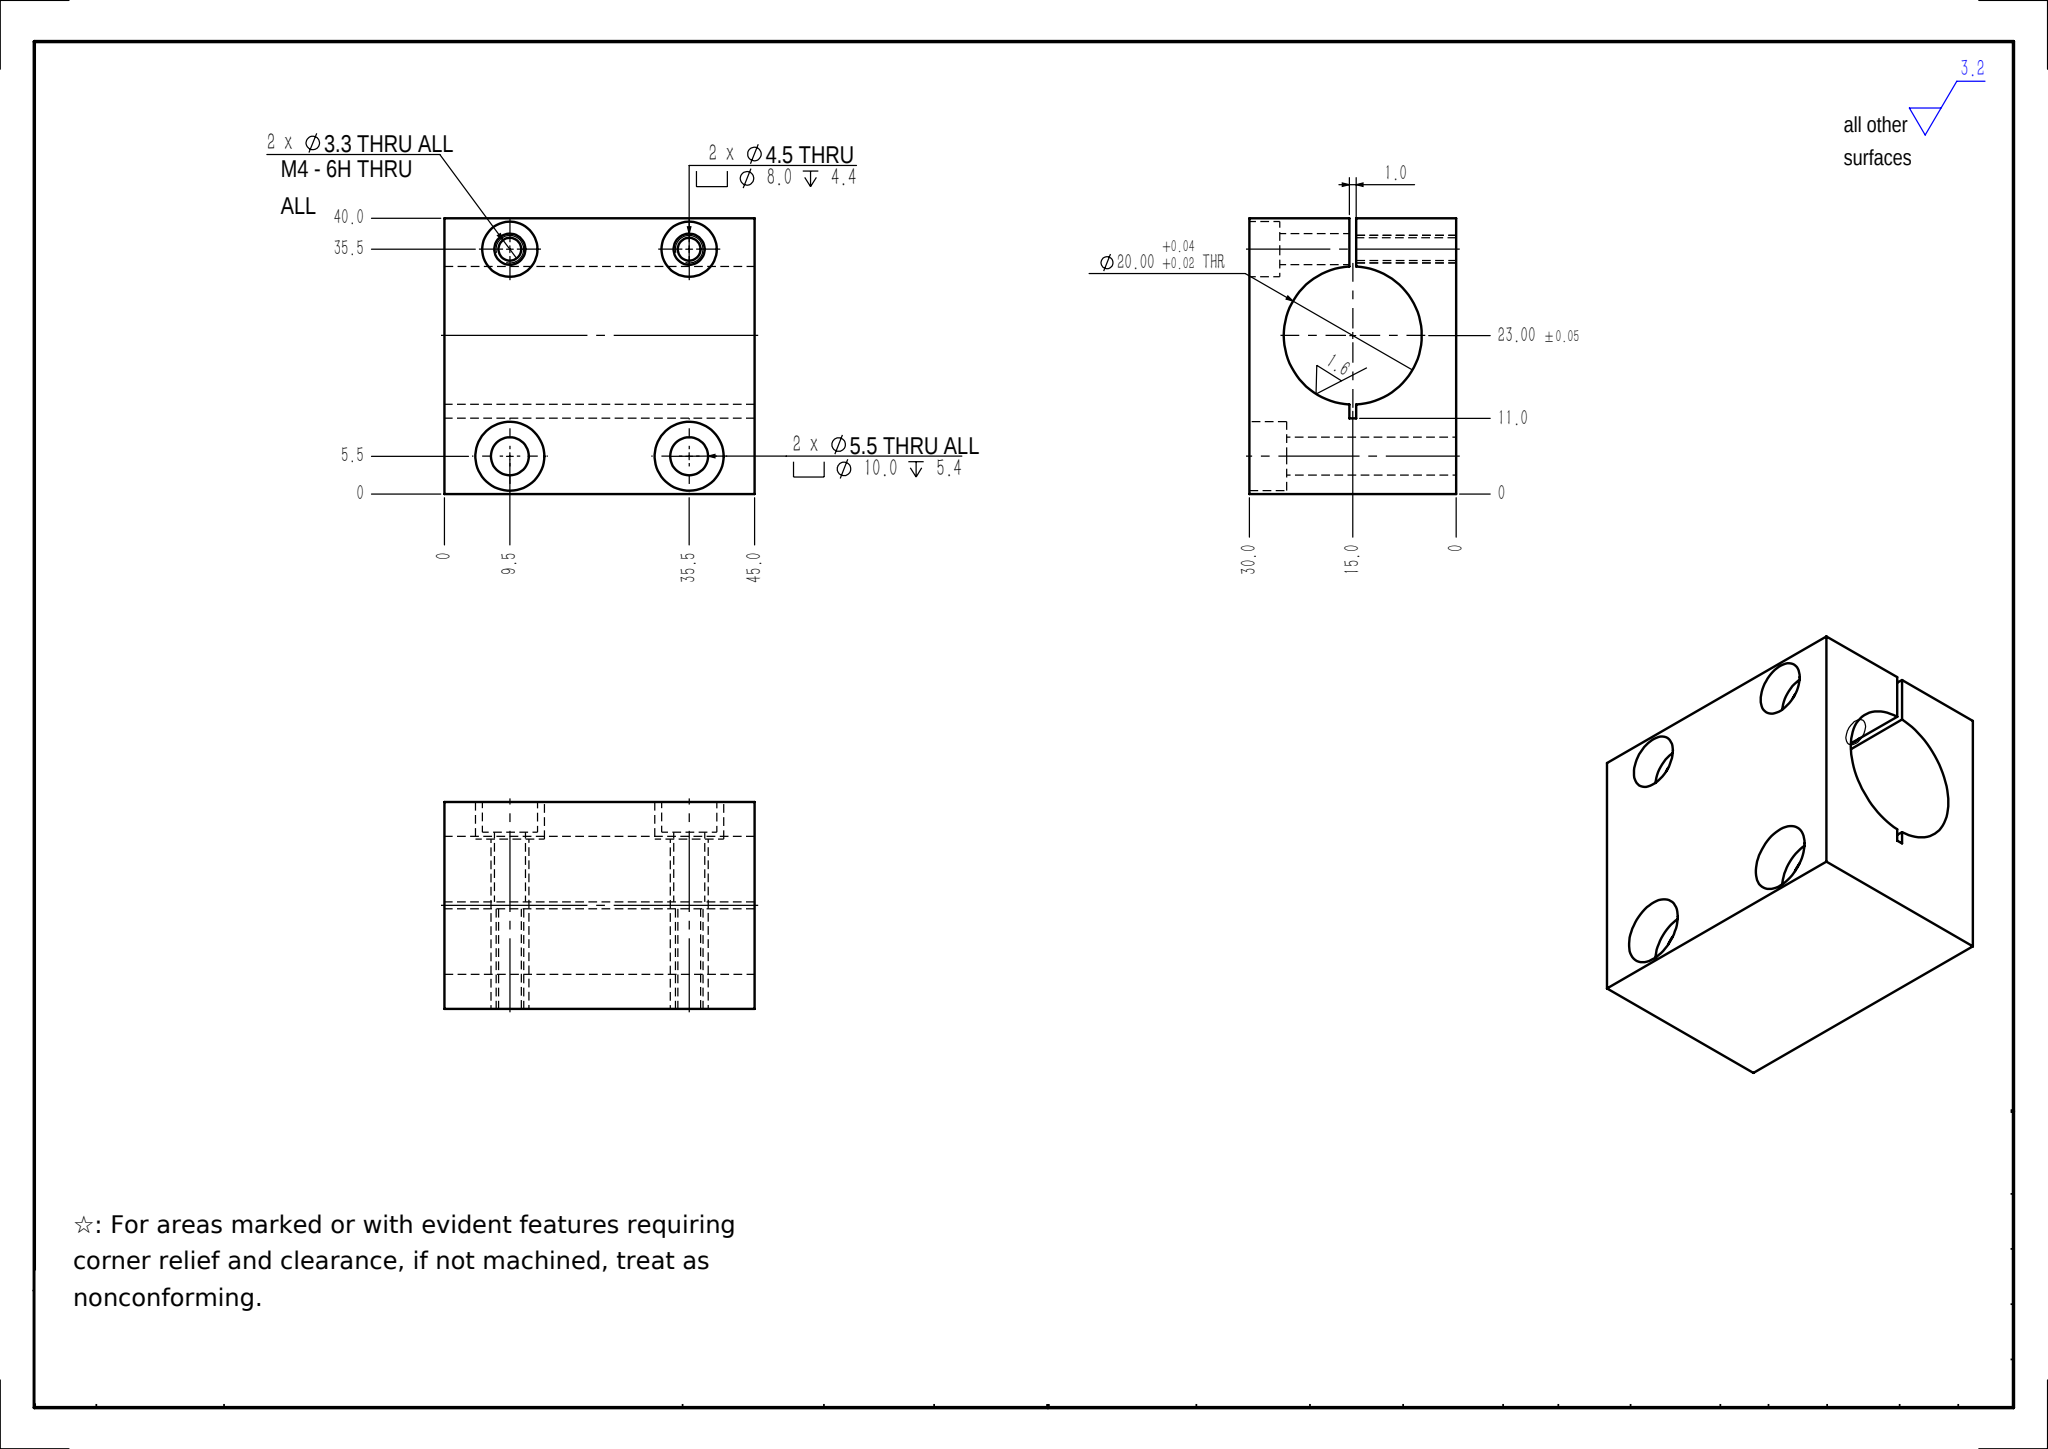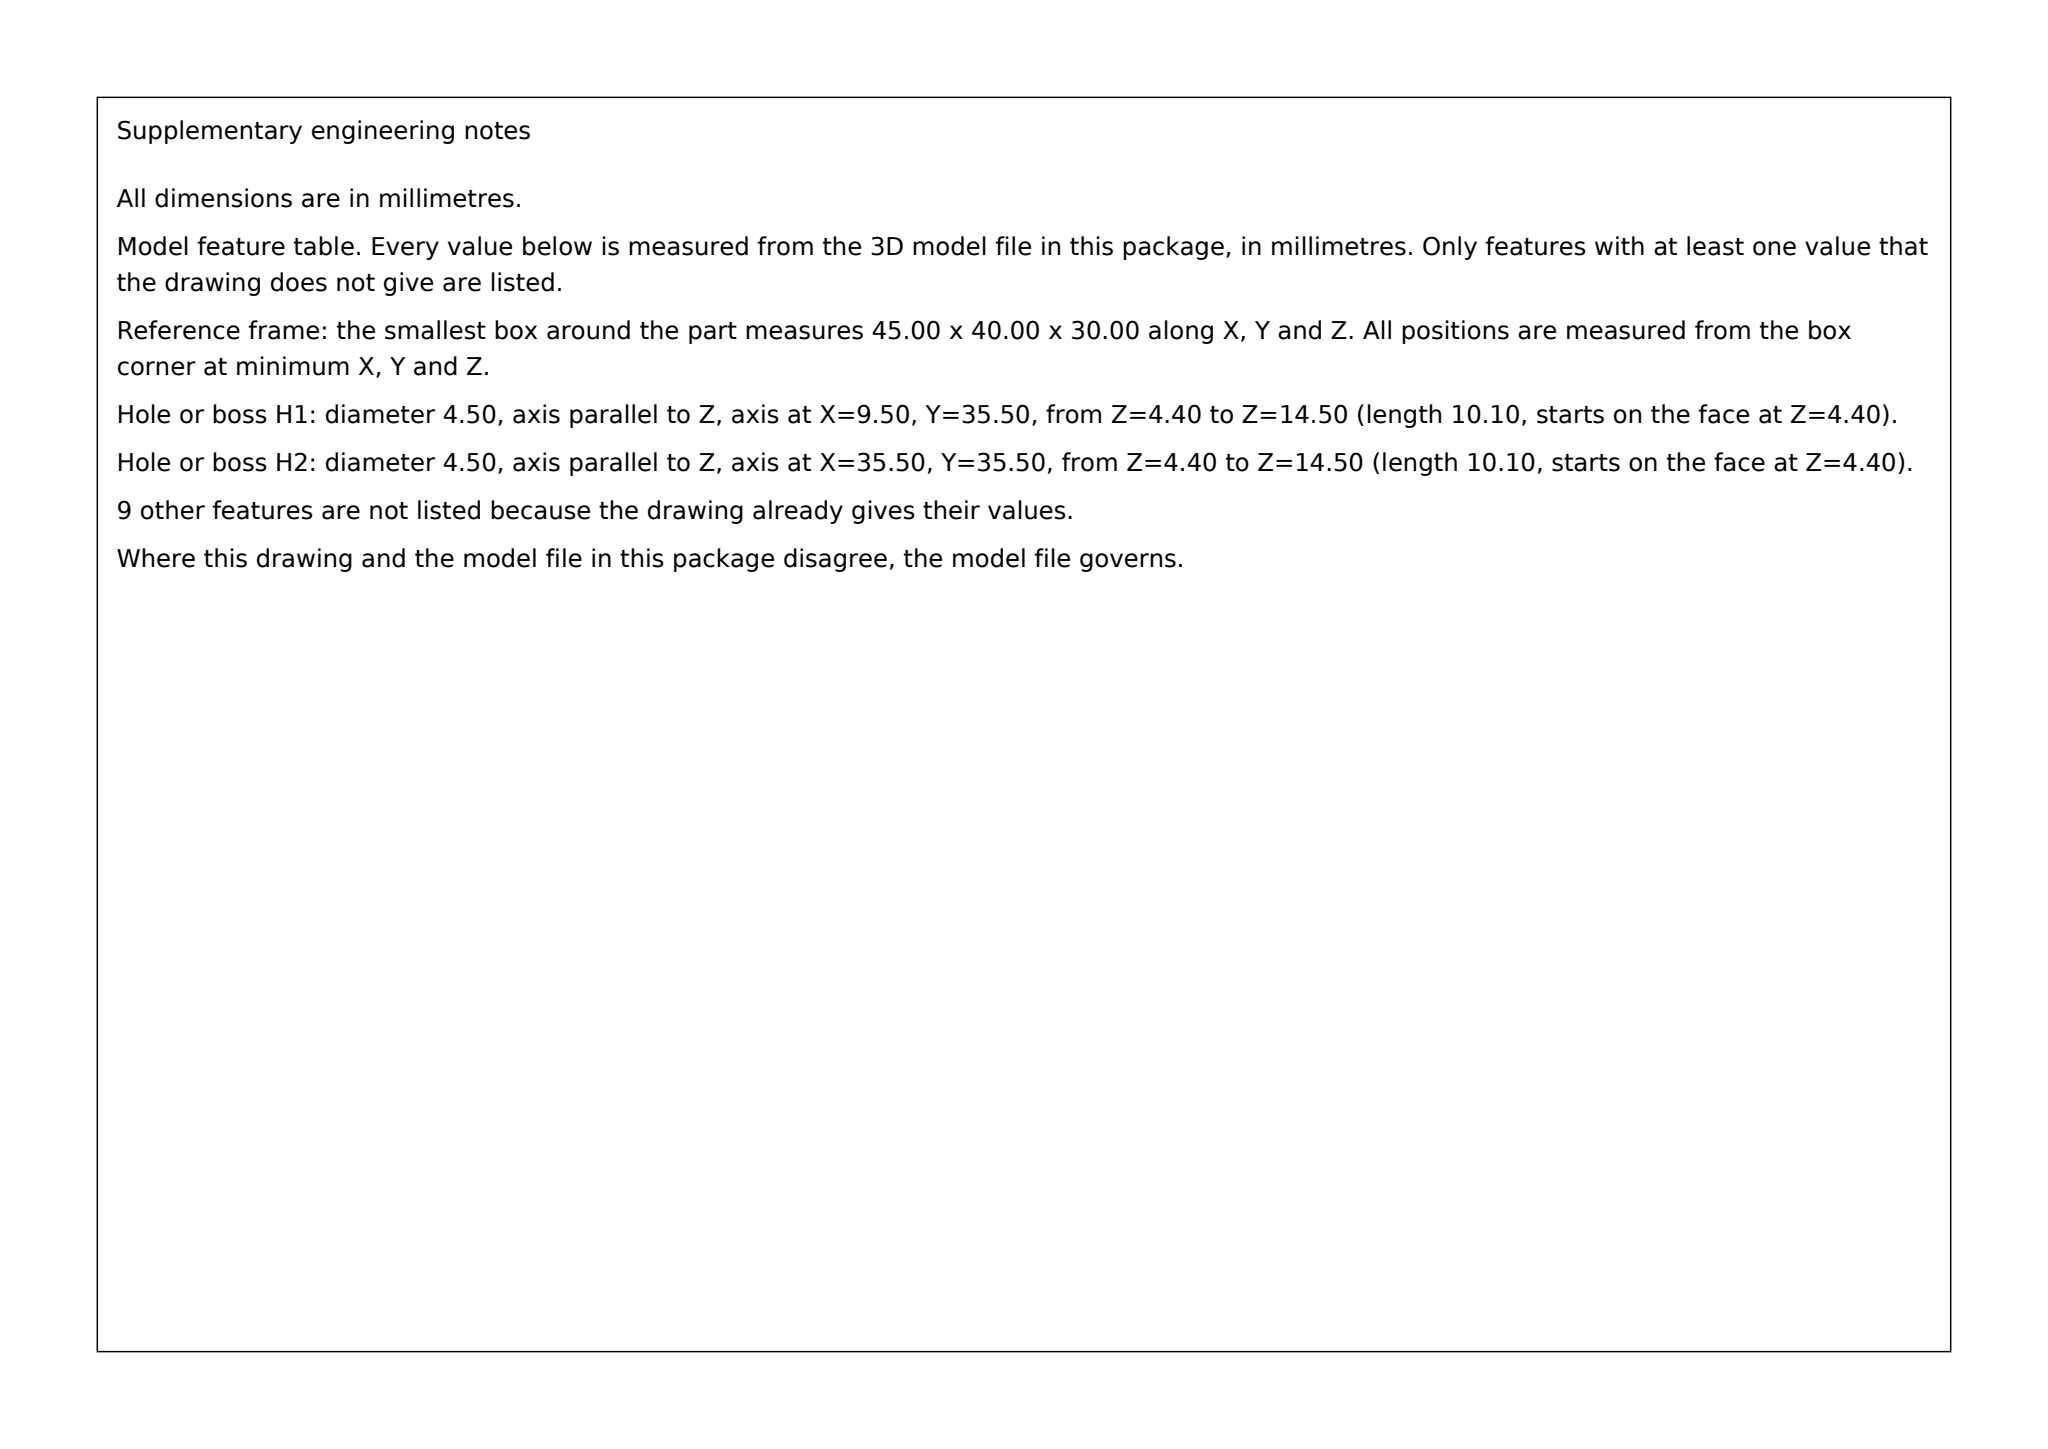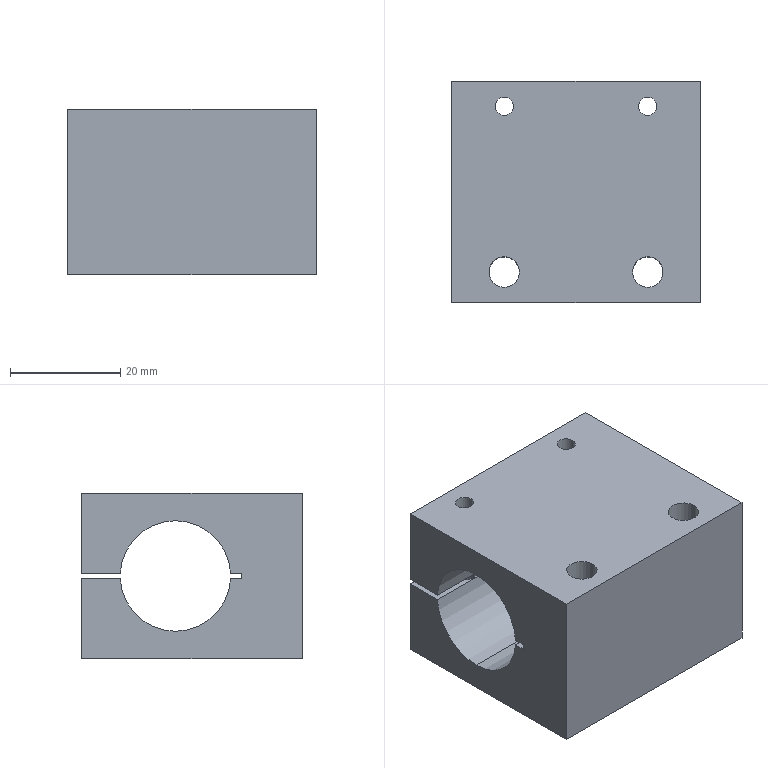Part | SolidWorks | mm | 1 solid | 39 faces | box 45 x 40 x 30 mm | volume 36429 mm3 | cylinder 23 | plane 16 | commonest cylinder face diameters 3.3 x4 8 x4 4.5 x4 10 x4 5.5 x4 20 x3
build123d program:
from build123d import *

# Parameters (mm, degrees)
SKETCH1_W                                       = 45
SKETCH1_H                                       = 40
BOSS_EXTRUDE1_DEPTH                             = 15
SKETCH2_R                                       = 10
CUT_EXTRUDE1_DEPTH                              = 52.478
SKETCH3_W                                       = 1
SKETCH3_H                                       = 29
CUT_EXTRUDE2_DEPTH                              = 52.478
M5_HEX_SOCKET_HEAD_CAP_SCREW_CBORE1_D           = 5.5
M5_HEX_SOCKET_HEAD_CAP_SCREW_CBORE1_CBORE_D     = 10
M5_HEX_SOCKET_HEAD_CAP_SCREW_CBORE1_CBORE_DEPTH = 5.4
M4_HEX_SOCKET_HEAD_CAP_SCREW_CBORE1_D           = 4.5
M4_HEX_SOCKET_HEAD_CAP_SCREW_CBORE1_DEPTH       = 14.5
M4_HEX_SOCKET_HEAD_CAP_SCREW_CBORE1_CBORE_D     = 8
M4_HEX_SOCKET_HEAD_CAP_SCREW_CBORE1_CBORE_DEPTH = 4.4
M4_TAPPED_HOLE1_D                               = 3.3


with BuildPart() as part:
    # Sketch1 → Boss-Extrude1 (new, symmetric)
    with BuildSketch(Plane.XY):
        Rectangle(SKETCH1_W, SKETCH1_H)
    extrude(amount=BOSS_EXTRUDE1_DEPTH, both=True)

    # Sketch2 → Cut-Extrude1 (cut, through all)
    with BuildSketch(Plane(origin=(22.5, 0, 0), x_dir=(0, 0, -1), z_dir=(1, 0, 0))):
        with Locations((0, 3)):
            Circle(SKETCH2_R)
    extrude(amount=-CUT_EXTRUDE1_DEPTH, mode=Mode.SUBTRACT)

    # Sketch3 → Cut-Extrude2 (cut, through all)
    with BuildSketch(Plane(origin=(22.5, 0, 0), x_dir=(0, 0, -1), z_dir=(1, 0, 0))):
        with Locations((0, 5.5)):
            Rectangle(SKETCH3_W, SKETCH3_H)
    extrude(amount=-CUT_EXTRUDE2_DEPTH, mode=Mode.SUBTRACT)

    # M5 Hex Socket Head Cap Screw CBORE1 (through all)
    with Locations(Plane(origin=(0, 0, -15), x_dir=(-1, 0, 0), z_dir=(0, 0, -1))):
        with Locations((-13, -14.5), (13, -14.5)):
            CounterBoreHole(M5_HEX_SOCKET_HEAD_CAP_SCREW_CBORE1_D / 2, M5_HEX_SOCKET_HEAD_CAP_SCREW_CBORE1_CBORE_D / 2, M5_HEX_SOCKET_HEAD_CAP_SCREW_CBORE1_CBORE_DEPTH)

    # M4 Hex Socket Head Cap Screw CBORE1
    with Locations(Plane(origin=(0, 0, -15), x_dir=(-1, 0, 0), z_dir=(0, 0, -1))):
        with Locations((-13, 15.5), (13, 15.5)):
            CounterBoreHole(M4_HEX_SOCKET_HEAD_CAP_SCREW_CBORE1_D / 2, M4_HEX_SOCKET_HEAD_CAP_SCREW_CBORE1_CBORE_D / 2, M4_HEX_SOCKET_HEAD_CAP_SCREW_CBORE1_CBORE_DEPTH, depth=M4_HEX_SOCKET_HEAD_CAP_SCREW_CBORE1_DEPTH)

    # M4 Tapped Hole1 (through all)
    with Locations(Plane(origin=(0, 0, 0.5), x_dir=(-1, 0, 0), z_dir=(0, 0, -1))):
        with Locations((-13, 15.5), (13, 15.5)):
            Hole(M4_TAPPED_HOLE1_D / 2)


solid = part.part